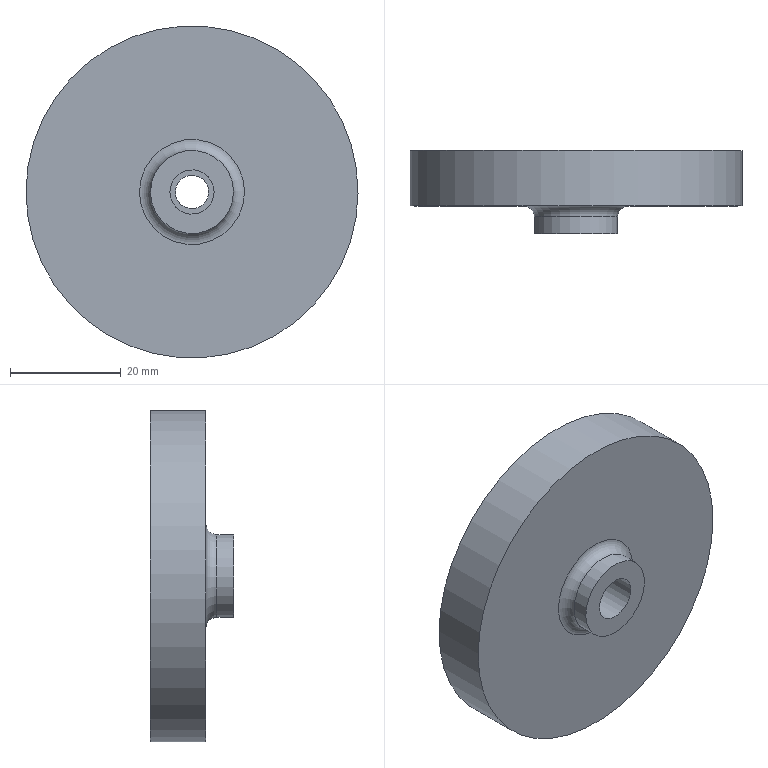Component | NX | PULLEY | 1 solid | 16 faces | box 60 x 15 x 60 mm | volume 22186 mm3 | plane 6 | cylinder 4 | torus 4 | cone 2 | commonest cylinder face diameters 15 x1 60 x1 8 x1 6 x1
STEP:
#1=CARTESIAN_POINT('',(0.,0.,0.));
#2=DIRECTION('',(0.,0.,1.));
#3=DIRECTION('',(1.,0.,0.));
#4=AXIS2_PLACEMENT_3D('',#1,#2,#3);
#5=CARTESIAN_POINT('',(-2.69,59.8,44.627));
#6=VERTEX_POINT('',#5);
#7=CARTESIAN_POINT('',(0.0005589,59.8,43.3));
#8=DIRECTION('',(0.,-1.,0.));
#9=DIRECTION('',(-0.8969,0.,0.4423));
#10=AXIS2_PLACEMENT_3D('',#7,#8,#9);
#11=CIRCLE('',#10,3.);
#12=CARTESIAN_POINT('',(0.0005589,59.8,43.3));
#13=DIRECTION('',(0.,1.,0.));
#14=DIRECTION('',(-0.8969,0.,0.4423));
#15=AXIS2_PLACEMENT_3D('',#12,#13,#14);
#16=PLANE('',#15);
#17=CARTESIAN_POINT('',(3.,-0.));
#18=CARTESIAN_POINT('',(3.,-5.196));
#19=CARTESIAN_POINT('',(-1.5,-2.598));
#20=CARTESIAN_POINT('',(-6.,0.));
#21=CARTESIAN_POINT('',(-1.5,2.598));
#22=CARTESIAN_POINT('',(3.,5.196));
#23=CARTESIAN_POINT('',(3.,-0.));
#24=(BOUNDED_CURVE()B_SPLINE_CURVE(2,(#17,#18,#19,#20,#21,#22,#23),.UNSPECIFIED.,.T.,.F.)B_SPLINE_CURVE_WITH_KNOTS((1,2,2,2,2,1),(-2.094,0.,2.094,4.189,6.283,8.378),.UNSPECIFIED.)CURVE()GEOMETRIC_REPRESENTATION_ITEM()RATIONAL_B_SPLINE_CURVE((1.,0.5,1.,0.5,1.,0.5,1.))REPRESENTATION_ITEM(''));
#25=(GEOMETRIC_REPRESENTATION_CONTEXT(2)PARAMETRIC_REPRESENTATION_CONTEXT()REPRESENTATION_CONTEXT('',''));
#26=DEFINITIONAL_REPRESENTATION('',(#24),#25);
#27=PCURVE('',#16,#26);
#28=CARTESIAN_POINT('',(0.0005589,73.3,43.3));
#29=DIRECTION('',(0.,-1.,0.));
#30=DIRECTION('',(0.8969,0.,-0.4423));
#31=AXIS2_PLACEMENT_3D('',#28,#29,#30);
#32=CYLINDRICAL_SURFACE('',#31,3.);
#33=CARTESIAN_POINT('',(3.142,13.5));
#34=DIRECTION('',(1.,0.));
#35=VECTOR('',#34,1.);
#36=LINE('',#33,#35);
#37=(GEOMETRIC_REPRESENTATION_CONTEXT(2)PARAMETRIC_REPRESENTATION_CONTEXT()REPRESENTATION_CONTEXT('',''));
#38=DEFINITIONAL_REPRESENTATION('',(#36),#37);
#39=PCURVE('',#32,#38);
#40=SURFACE_CURVE('',#11,(#27,#39),.PCURVE_S1.);
#41=EDGE_CURVE('',#6,#6,#40,.T.);
#42=ORIENTED_EDGE('',*,*,#41,.T.);
#43=EDGE_LOOP('',(#42));
#44=FACE_BOUND('',#43,.T.);
#45=CARTESIAN_POINT('',(5.382,59.8,40.646));
#46=VERTEX_POINT('',#45);
#47=CARTESIAN_POINT('',(0.0005589,59.8,43.3));
#48=DIRECTION('',(0.,-1.,0.));
#49=DIRECTION('',(0.8969,0.,-0.4423));
#50=AXIS2_PLACEMENT_3D('',#47,#48,#49);
#51=CIRCLE('',#50,6.);
#52=CARTESIAN_POINT('',(-6.,0.));
#53=CARTESIAN_POINT('',(-6.,10.392));
#54=CARTESIAN_POINT('',(3.,5.196));
#55=CARTESIAN_POINT('',(12.,0.));
#56=CARTESIAN_POINT('',(3.,-5.196));
#57=CARTESIAN_POINT('',(-6.,-10.392));
#58=CARTESIAN_POINT('',(-6.,0.));
#59=(BOUNDED_CURVE()B_SPLINE_CURVE(2,(#52,#53,#54,#55,#56,#57,#58),.UNSPECIFIED.,.T.,.F.)B_SPLINE_CURVE_WITH_KNOTS((1,2,2,2,2,1),(-2.094,0.,2.094,4.189,6.283,8.378),.UNSPECIFIED.)CURVE()GEOMETRIC_REPRESENTATION_ITEM()RATIONAL_B_SPLINE_CURVE((1.,0.5,1.,0.5,1.,0.5,1.))REPRESENTATION_ITEM(''));
#60=(GEOMETRIC_REPRESENTATION_CONTEXT(2)PARAMETRIC_REPRESENTATION_CONTEXT()REPRESENTATION_CONTEXT('',''));
#61=DEFINITIONAL_REPRESENTATION('',(#59),#60);
#62=PCURVE('',#16,#61);
#63=CARTESIAN_POINT('',(0.0005589,53.8,43.3));
#64=DIRECTION('',(0.,-1.,0.));
#65=DIRECTION('',(0.8969,0.,-0.4423));
#66=AXIS2_PLACEMENT_3D('',#63,#64,#65);
#67=CONICAL_SURFACE('',#66,6.843,0.1396);
#68=CARTESIAN_POINT('',(0.,-6.));
#69=DIRECTION('',(1.,-0.));
#70=VECTOR('',#69,1.);
#71=LINE('',#68,#70);
#72=(GEOMETRIC_REPRESENTATION_CONTEXT(2)PARAMETRIC_REPRESENTATION_CONTEXT()REPRESENTATION_CONTEXT('',''));
#73=DEFINITIONAL_REPRESENTATION('',(#71),#72);
#74=PCURVE('',#67,#73);
#75=SURFACE_CURVE('',#51,(#62,#74),.PCURVE_S1.);
#76=EDGE_CURVE('',#46,#46,#75,.T.);
#77=ORIENTED_EDGE('',*,*,#76,.F.);
#78=EDGE_LOOP('',(#77));
#79=FACE_BOUND('',#78,.T.);
#80=ADVANCED_FACE('',(#44,#79),#16,.T.);
#81=CARTESIAN_POINT('',(-3.587,44.8,45.069));
#82=VERTEX_POINT('',#81);
#83=CARTESIAN_POINT('',(0.0005589,44.8,43.3));
#84=DIRECTION('',(0.,1.,0.));
#85=DIRECTION('',(-0.8969,0.,0.4423));
#86=AXIS2_PLACEMENT_3D('',#83,#84,#85);
#87=CIRCLE('',#86,4.);
#88=CARTESIAN_POINT('',(0.0005589,44.8,43.3));
#89=DIRECTION('',(0.,-1.,0.));
#90=DIRECTION('',(0.8969,0.,-0.4423));
#91=AXIS2_PLACEMENT_3D('',#88,#89,#90);
#92=PLANE('',#91);
#93=CARTESIAN_POINT('',(-4.,0.));
#94=CARTESIAN_POINT('',(-4.,6.928));
#95=CARTESIAN_POINT('',(2.,3.464));
#96=CARTESIAN_POINT('',(8.,0.));
#97=CARTESIAN_POINT('',(2.,-3.464));
#98=CARTESIAN_POINT('',(-4.,-6.928));
#99=CARTESIAN_POINT('',(-4.,0.));
#100=(BOUNDED_CURVE()B_SPLINE_CURVE(2,(#93,#94,#95,#96,#97,#98,#99),.UNSPECIFIED.,.T.,.F.)B_SPLINE_CURVE_WITH_KNOTS((1,2,2,2,2,1),(-2.094,0.,2.094,4.189,6.283,8.378),.UNSPECIFIED.)CURVE()GEOMETRIC_REPRESENTATION_ITEM()RATIONAL_B_SPLINE_CURVE((1.,0.5,1.,0.5,1.,0.5,1.))REPRESENTATION_ITEM(''));
#101=(GEOMETRIC_REPRESENTATION_CONTEXT(2)PARAMETRIC_REPRESENTATION_CONTEXT()REPRESENTATION_CONTEXT('',''));
#102=DEFINITIONAL_REPRESENTATION('',(#100),#101);
#103=PCURVE('',#92,#102);
#104=CARTESIAN_POINT('',(0.0005589,52.3,43.3));
#105=DIRECTION('',(0.,-1.,0.));
#106=DIRECTION('',(0.8969,0.,-0.4423));
#107=AXIS2_PLACEMENT_3D('',#104,#105,#106);
#108=CYLINDRICAL_SURFACE('',#107,4.);
#109=CARTESIAN_POINT('',(9.425,7.5));
#110=DIRECTION('',(-1.,0.));
#111=VECTOR('',#110,1.);
#112=LINE('',#109,#111);
#113=(GEOMETRIC_REPRESENTATION_CONTEXT(2)PARAMETRIC_REPRESENTATION_CONTEXT()REPRESENTATION_CONTEXT('',''));
#114=DEFINITIONAL_REPRESENTATION('',(#112),#113);
#115=PCURVE('',#108,#114);
#116=SURFACE_CURVE('',#87,(#103,#115),.PCURVE_S1.);
#117=EDGE_CURVE('',#82,#82,#116,.T.);
#118=ORIENTED_EDGE('',*,*,#117,.T.);
#119=EDGE_LOOP('',(#118));
#120=FACE_BOUND('',#119,.T.);
#121=CARTESIAN_POINT('',(-6.726,44.8,46.617));
#122=VERTEX_POINT('',#121);
#123=CARTESIAN_POINT('',(0.0005589,44.8,43.3));
#124=DIRECTION('',(0.,1.,0.));
#125=DIRECTION('',(-0.8969,0.,0.4423));
#126=AXIS2_PLACEMENT_3D('',#123,#124,#125);
#127=CIRCLE('',#126,7.5);
#128=CARTESIAN_POINT('',(-7.5,0.));
#129=CARTESIAN_POINT('',(-7.5,12.99));
#130=CARTESIAN_POINT('',(3.75,6.495));
#131=CARTESIAN_POINT('',(15.,0.));
#132=CARTESIAN_POINT('',(3.75,-6.495));
#133=CARTESIAN_POINT('',(-7.5,-12.99));
#134=CARTESIAN_POINT('',(-7.5,0.));
#135=(BOUNDED_CURVE()B_SPLINE_CURVE(2,(#128,#129,#130,#131,#132,#133,#134),.UNSPECIFIED.,.T.,.F.)B_SPLINE_CURVE_WITH_KNOTS((1,2,2,2,2,1),(-2.094,0.,2.094,4.189,6.283,8.378),.UNSPECIFIED.)CURVE()GEOMETRIC_REPRESENTATION_ITEM()RATIONAL_B_SPLINE_CURVE((1.,0.5,1.,0.5,1.,0.5,1.))REPRESENTATION_ITEM(''));
#136=(GEOMETRIC_REPRESENTATION_CONTEXT(2)PARAMETRIC_REPRESENTATION_CONTEXT()REPRESENTATION_CONTEXT('',''));
#137=DEFINITIONAL_REPRESENTATION('',(#135),#136);
#138=PCURVE('',#92,#137);
#139=CARTESIAN_POINT('',(0.0005589,44.8,43.3));
#140=DIRECTION('',(0.,1.,0.));
#141=DIRECTION('',(-0.8969,0.,0.4423));
#142=AXIS2_PLACEMENT_3D('',#139,#140,#141);
#143=CYLINDRICAL_SURFACE('',#142,7.5);
#144=CARTESIAN_POINT('',(0.,0.));
#145=DIRECTION('',(1.,0.));
#146=VECTOR('',#145,1.);
#147=LINE('',#144,#146);
#148=(GEOMETRIC_REPRESENTATION_CONTEXT(2)PARAMETRIC_REPRESENTATION_CONTEXT()REPRESENTATION_CONTEXT('',''));
#149=DEFINITIONAL_REPRESENTATION('',(#147),#148);
#150=PCURVE('',#143,#149);
#151=SURFACE_CURVE('',#127,(#138,#150),.PCURVE_S1.);
#152=EDGE_CURVE('',#122,#122,#151,.T.);
#153=ORIENTED_EDGE('',*,*,#152,.F.);
#154=EDGE_LOOP('',(#153));
#155=FACE_BOUND('',#154,.T.);
#156=ADVANCED_FACE('',(#120,#155),#92,.T.);
#157=CARTESIAN_POINT('',(6.727,47.8,39.983));
#158=VERTEX_POINT('',#157);
#159=CARTESIAN_POINT('',(-6.726,47.8,46.617));
#160=VERTEX_POINT('',#159);
#161=CARTESIAN_POINT('',(0.0005589,47.8,43.3));
#162=DIRECTION('',(0.,-1.,0.));
#163=DIRECTION('',(0.8969,0.,-0.4423));
#164=AXIS2_PLACEMENT_3D('',#161,#162,#163);
#165=CIRCLE('',#164,7.5);
#166=CARTESIAN_POINT('',(3.142,3.));
#167=DIRECTION('',(-1.,0.));
#168=VECTOR('',#167,1.);
#169=LINE('',#166,#168);
#170=(GEOMETRIC_REPRESENTATION_CONTEXT(2)PARAMETRIC_REPRESENTATION_CONTEXT()REPRESENTATION_CONTEXT('',''));
#171=DEFINITIONAL_REPRESENTATION('',(#169),#170);
#172=PCURVE('',#143,#171);
#173=CARTESIAN_POINT('',(0.0005589,47.8,43.3));
#174=DIRECTION('',(0.,-1.,0.));
#175=DIRECTION('',(0.8969,0.,-0.4423));
#176=AXIS2_PLACEMENT_3D('',#173,#174,#175);
#177=TOROIDAL_SURFACE('',#176,9.5,2.);
#178=CARTESIAN_POINT('',(0.,3.142));
#179=DIRECTION('',(1.,-0.));
#180=VECTOR('',#179,1.);
#181=LINE('',#178,#180);
#182=(GEOMETRIC_REPRESENTATION_CONTEXT(2)PARAMETRIC_REPRESENTATION_CONTEXT()REPRESENTATION_CONTEXT('',''));
#183=DEFINITIONAL_REPRESENTATION('',(#181),#182);
#184=PCURVE('',#177,#183);
#185=SURFACE_CURVE('',#165,(#172,#184),.PCURVE_S1.);
#186=EDGE_CURVE('',#158,#160,#185,.T.);
#187=ORIENTED_EDGE('',*,*,#186,.T.);
#188=CARTESIAN_POINT('',(-6.726,44.8,46.617));
#189=CARTESIAN_POINT('',(-6.726,47.8,46.617));
#190=B_SPLINE_CURVE_WITH_KNOTS('',1,(#188,#189),.UNSPECIFIED.,.F.,.F.,(2,2),(0.,3.),.PIECEWISE_BEZIER_KNOTS.);
#191=CARTESIAN_POINT('',(0.,0.));
#192=DIRECTION('',(0.,1.));
#193=VECTOR('',#192,1.);
#194=LINE('',#191,#193);
#195=(GEOMETRIC_REPRESENTATION_CONTEXT(2)PARAMETRIC_REPRESENTATION_CONTEXT()REPRESENTATION_CONTEXT('',''));
#196=DEFINITIONAL_REPRESENTATION('',(#194),#195);
#197=PCURVE('',#143,#196);
#198=CARTESIAN_POINT('',(6.283,0.));
#199=DIRECTION('',(0.,1.));
#200=VECTOR('',#199,1.);
#201=LINE('',#198,#200);
#202=(GEOMETRIC_REPRESENTATION_CONTEXT(2)PARAMETRIC_REPRESENTATION_CONTEXT()REPRESENTATION_CONTEXT('',''));
#203=DEFINITIONAL_REPRESENTATION('',(#201),#202);
#204=PCURVE('',#143,#203);
#205=SEAM_CURVE('',#190,(#197,#204),.PCURVE_S1.);
#206=EDGE_CURVE('',#122,#160,#205,.T.);
#207=ORIENTED_EDGE('',*,*,#206,.F.);
#208=ORIENTED_EDGE('',*,*,#152,.T.);
#209=ORIENTED_EDGE('',*,*,#206,.T.);
#210=CARTESIAN_POINT('',(0.0005589,47.8,43.3));
#211=DIRECTION('',(0.,-1.,0.));
#212=DIRECTION('',(0.8969,0.,-0.4423));
#213=AXIS2_PLACEMENT_3D('',#210,#211,#212);
#214=CIRCLE('',#213,7.5);
#215=CARTESIAN_POINT('',(9.425,3.));
#216=DIRECTION('',(-1.,0.));
#217=VECTOR('',#216,1.);
#218=LINE('',#215,#217);
#219=(GEOMETRIC_REPRESENTATION_CONTEXT(2)PARAMETRIC_REPRESENTATION_CONTEXT()REPRESENTATION_CONTEXT('',''));
#220=DEFINITIONAL_REPRESENTATION('',(#218),#219);
#221=PCURVE('',#143,#220);
#222=CARTESIAN_POINT('',(0.,3.142));
#223=DIRECTION('',(1.,0.));
#224=VECTOR('',#223,1.);
#225=LINE('',#222,#224);
#226=(GEOMETRIC_REPRESENTATION_CONTEXT(2)PARAMETRIC_REPRESENTATION_CONTEXT()REPRESENTATION_CONTEXT('',''));
#227=DEFINITIONAL_REPRESENTATION('',(#225),#226);
#228=PCURVE('',#177,#227);
#229=SURFACE_CURVE('',#214,(#221,#228),.PCURVE_S1.);
#230=EDGE_CURVE('',#160,#158,#229,.T.);
#231=ORIENTED_EDGE('',*,*,#230,.T.);
#232=EDGE_LOOP('',(#187,#207,#208,#209,#231));
#233=FACE_BOUND('',#232,.T.);
#234=ADVANCED_FACE('',(#233),#143,.T.);
#235=CARTESIAN_POINT('',(-18.907,59.8,52.624));
#236=VERTEX_POINT('',#235);
#237=CARTESIAN_POINT('',(0.0005589,59.8,43.3));
#238=DIRECTION('',(0.,-1.,0.));
#239=DIRECTION('',(-0.8969,0.,0.4423));
#240=AXIS2_PLACEMENT_3D('',#237,#238,#239);
#241=CIRCLE('',#240,21.081);
#242=CARTESIAN_POINT('',(0.0005589,59.8,43.3));
#243=DIRECTION('',(0.,1.,0.));
#244=DIRECTION('',(-0.8969,0.,0.4423));
#245=AXIS2_PLACEMENT_3D('',#242,#243,#244);
#246=PLANE('',#245);
#247=CARTESIAN_POINT('',(21.081,0.));
#248=CARTESIAN_POINT('',(21.081,-36.514));
#249=CARTESIAN_POINT('',(-10.541,-18.257));
#250=CARTESIAN_POINT('',(-42.163,-0.));
#251=CARTESIAN_POINT('',(-10.541,18.257));
#252=CARTESIAN_POINT('',(21.081,36.514));
#253=CARTESIAN_POINT('',(21.081,0.));
#254=(BOUNDED_CURVE()B_SPLINE_CURVE(2,(#247,#248,#249,#250,#251,#252,#253),.UNSPECIFIED.,.T.,.F.)B_SPLINE_CURVE_WITH_KNOTS((1,2,2,2,2,1),(-2.094,0.,2.094,4.189,6.283,8.378),.UNSPECIFIED.)CURVE()GEOMETRIC_REPRESENTATION_ITEM()RATIONAL_B_SPLINE_CURVE((1.,0.5,1.,0.5,1.,0.5,1.))REPRESENTATION_ITEM(''));
#255=(GEOMETRIC_REPRESENTATION_CONTEXT(2)PARAMETRIC_REPRESENTATION_CONTEXT()REPRESENTATION_CONTEXT('',''));
#256=DEFINITIONAL_REPRESENTATION('',(#254),#255);
#257=PCURVE('',#246,#256);
#258=CARTESIAN_POINT('',(0.0005589,58.8,43.3));
#259=DIRECTION('',(0.,1.,0.));
#260=DIRECTION('',(-0.8969,0.,0.4423));
#261=AXIS2_PLACEMENT_3D('',#258,#259,#260);
#262=TOROIDAL_SURFACE('',#261,21.081,1.);
#263=CARTESIAN_POINT('',(6.283,7.854));
#264=DIRECTION('',(-1.,0.));
#265=VECTOR('',#264,1.);
#266=LINE('',#263,#265);
#267=(GEOMETRIC_REPRESENTATION_CONTEXT(2)PARAMETRIC_REPRESENTATION_CONTEXT()REPRESENTATION_CONTEXT('',''));
#268=DEFINITIONAL_REPRESENTATION('',(#266),#267);
#269=PCURVE('',#262,#268);
#270=SURFACE_CURVE('',#241,(#257,#269),.PCURVE_S1.);
#271=EDGE_CURVE('',#236,#236,#270,.T.);
#272=ORIENTED_EDGE('',*,*,#271,.T.);
#273=EDGE_LOOP('',(#272));
#274=FACE_BOUND('',#273,.T.);
#275=CARTESIAN_POINT('',(-26.906,59.8,56.569));
#276=VERTEX_POINT('',#275);
#277=CARTESIAN_POINT('',(0.0005589,59.8,43.3));
#278=DIRECTION('',(0.,1.,0.));
#279=DIRECTION('',(-0.8969,0.,0.4423));
#280=AXIS2_PLACEMENT_3D('',#277,#278,#279);
#281=CIRCLE('',#280,30.);
#282=CARTESIAN_POINT('',(0.,0.));
#283=DIRECTION('',(1.,0.));
#284=AXIS2_PLACEMENT_2D('',#282,#283);
#285=CIRCLE('',#284,30.);
#286=(GEOMETRIC_REPRESENTATION_CONTEXT(2)PARAMETRIC_REPRESENTATION_CONTEXT()REPRESENTATION_CONTEXT('',''));
#287=DEFINITIONAL_REPRESENTATION('',(#285),#286);
#288=PCURVE('',#246,#287);
#289=CARTESIAN_POINT('',(0.0005589,49.8,43.3));
#290=DIRECTION('',(0.,1.,0.));
#291=DIRECTION('',(-0.8969,0.,0.4423));
#292=AXIS2_PLACEMENT_3D('',#289,#290,#291);
#293=CYLINDRICAL_SURFACE('',#292,30.);
#294=CARTESIAN_POINT('',(0.,10.));
#295=DIRECTION('',(1.,0.));
#296=VECTOR('',#295,1.);
#297=LINE('',#294,#296);
#298=(GEOMETRIC_REPRESENTATION_CONTEXT(2)PARAMETRIC_REPRESENTATION_CONTEXT()REPRESENTATION_CONTEXT('',''));
#299=DEFINITIONAL_REPRESENTATION('',(#297),#298);
#300=PCURVE('',#293,#299);
#301=SURFACE_CURVE('',#281,(#288,#300),.PCURVE_S1.);
#302=EDGE_CURVE('',#276,#276,#301,.T.);
#303=ORIENTED_EDGE('',*,*,#302,.T.);
#304=EDGE_LOOP('',(#303));
#305=FACE_BOUND('',#304,.T.);
#306=ADVANCED_FACE('',(#274,#305),#246,.T.);
#307=CARTESIAN_POINT('',(8.521,49.8,39.098));
#308=VERTEX_POINT('',#307);
#309=CARTESIAN_POINT('',(0.0005589,49.8,43.3));
#310=DIRECTION('',(0.,1.,0.));
#311=DIRECTION('',(0.8969,0.,-0.4423));
#312=AXIS2_PLACEMENT_3D('',#309,#310,#311);
#313=CIRCLE('',#312,9.5);
#314=CARTESIAN_POINT('',(0.0005589,49.8,43.3));
#315=DIRECTION('',(0.,-1.,0.));
#316=DIRECTION('',(0.8969,0.,-0.4423));
#317=AXIS2_PLACEMENT_3D('',#314,#315,#316);
#318=PLANE('',#317);
#319=CARTESIAN_POINT('',(9.5,-0.));
#320=CARTESIAN_POINT('',(9.5,-16.454));
#321=CARTESIAN_POINT('',(-4.75,-8.227));
#322=CARTESIAN_POINT('',(-19.,0.));
#323=CARTESIAN_POINT('',(-4.75,8.227));
#324=CARTESIAN_POINT('',(9.5,16.454));
#325=CARTESIAN_POINT('',(9.5,-0.));
#326=(BOUNDED_CURVE()B_SPLINE_CURVE(2,(#319,#320,#321,#322,#323,#324,#325),.UNSPECIFIED.,.T.,.F.)B_SPLINE_CURVE_WITH_KNOTS((1,2,2,2,2,1),(-2.094,0.,2.094,4.189,6.283,8.378),.UNSPECIFIED.)CURVE()GEOMETRIC_REPRESENTATION_ITEM()RATIONAL_B_SPLINE_CURVE((1.,0.5,1.,0.5,1.,0.5,1.))REPRESENTATION_ITEM(''));
#327=(GEOMETRIC_REPRESENTATION_CONTEXT(2)PARAMETRIC_REPRESENTATION_CONTEXT()REPRESENTATION_CONTEXT('',''));
#328=DEFINITIONAL_REPRESENTATION('',(#326),#327);
#329=PCURVE('',#318,#328);
#330=CARTESIAN_POINT('',(6.283,4.712));
#331=DIRECTION('',(-1.,0.));
#332=VECTOR('',#331,1.);
#333=LINE('',#330,#332);
#334=(GEOMETRIC_REPRESENTATION_CONTEXT(2)PARAMETRIC_REPRESENTATION_CONTEXT()REPRESENTATION_CONTEXT('',''));
#335=DEFINITIONAL_REPRESENTATION('',(#333),#334);
#336=PCURVE('',#177,#335);
#337=SURFACE_CURVE('',#313,(#329,#336),.PCURVE_S1.);
#338=EDGE_CURVE('',#308,#308,#337,.T.);
#339=ORIENTED_EDGE('',*,*,#338,.T.);
#340=EDGE_LOOP('',(#339));
#341=FACE_BOUND('',#340,.T.);
#342=CARTESIAN_POINT('',(-26.906,49.8,56.569));
#343=VERTEX_POINT('',#342);
#344=CARTESIAN_POINT('',(0.0005589,49.8,43.3));
#345=DIRECTION('',(0.,1.,0.));
#346=DIRECTION('',(-0.8969,0.,0.4423));
#347=AXIS2_PLACEMENT_3D('',#344,#345,#346);
#348=CIRCLE('',#347,30.);
#349=CARTESIAN_POINT('',(-30.,0.));
#350=CARTESIAN_POINT('',(-30.,51.962));
#351=CARTESIAN_POINT('',(15.,25.981));
#352=CARTESIAN_POINT('',(60.,0.));
#353=CARTESIAN_POINT('',(15.,-25.981));
#354=CARTESIAN_POINT('',(-30.,-51.962));
#355=CARTESIAN_POINT('',(-30.,0.));
#356=(BOUNDED_CURVE()B_SPLINE_CURVE(2,(#349,#350,#351,#352,#353,#354,#355),.UNSPECIFIED.,.T.,.F.)B_SPLINE_CURVE_WITH_KNOTS((1,2,2,2,2,1),(-2.094,0.,2.094,4.189,6.283,8.378),.UNSPECIFIED.)CURVE()GEOMETRIC_REPRESENTATION_ITEM()RATIONAL_B_SPLINE_CURVE((1.,0.5,1.,0.5,1.,0.5,1.))REPRESENTATION_ITEM(''));
#357=(GEOMETRIC_REPRESENTATION_CONTEXT(2)PARAMETRIC_REPRESENTATION_CONTEXT()REPRESENTATION_CONTEXT('',''));
#358=DEFINITIONAL_REPRESENTATION('',(#356),#357);
#359=PCURVE('',#318,#358);
#360=CARTESIAN_POINT('',(0.,0.));
#361=DIRECTION('',(1.,0.));
#362=VECTOR('',#361,1.);
#363=LINE('',#360,#362);
#364=(GEOMETRIC_REPRESENTATION_CONTEXT(2)PARAMETRIC_REPRESENTATION_CONTEXT()REPRESENTATION_CONTEXT('',''));
#365=DEFINITIONAL_REPRESENTATION('',(#363),#364);
#366=PCURVE('',#293,#365);
#367=SURFACE_CURVE('',#348,(#359,#366),.PCURVE_S1.);
#368=EDGE_CURVE('',#343,#343,#367,.T.);
#369=ORIENTED_EDGE('',*,*,#368,.F.);
#370=EDGE_LOOP('',(#369));
#371=FACE_BOUND('',#370,.T.);
#372=ADVANCED_FACE('',(#341,#371),#318,.T.);
#373=ORIENTED_EDGE('',*,*,#302,.F.);
#374=CARTESIAN_POINT('',(-26.906,49.8,56.569));
#375=CARTESIAN_POINT('',(-26.906,59.8,56.569));
#376=B_SPLINE_CURVE_WITH_KNOTS('',1,(#374,#375),.UNSPECIFIED.,.F.,.F.,(2,2),(0.,10.),.PIECEWISE_BEZIER_KNOTS.);
#377=CARTESIAN_POINT('',(0.,0.));
#378=DIRECTION('',(0.,1.));
#379=VECTOR('',#378,1.);
#380=LINE('',#377,#379);
#381=(GEOMETRIC_REPRESENTATION_CONTEXT(2)PARAMETRIC_REPRESENTATION_CONTEXT()REPRESENTATION_CONTEXT('',''));
#382=DEFINITIONAL_REPRESENTATION('',(#380),#381);
#383=PCURVE('',#293,#382);
#384=CARTESIAN_POINT('',(6.283,0.));
#385=DIRECTION('',(0.,1.));
#386=VECTOR('',#385,1.);
#387=LINE('',#384,#386);
#388=(GEOMETRIC_REPRESENTATION_CONTEXT(2)PARAMETRIC_REPRESENTATION_CONTEXT()REPRESENTATION_CONTEXT('',''));
#389=DEFINITIONAL_REPRESENTATION('',(#387),#388);
#390=PCURVE('',#293,#389);
#391=SEAM_CURVE('',#376,(#383,#390),.PCURVE_S1.);
#392=EDGE_CURVE('',#343,#276,#391,.T.);
#393=ORIENTED_EDGE('',*,*,#392,.F.);
#394=ORIENTED_EDGE('',*,*,#368,.T.);
#395=ORIENTED_EDGE('',*,*,#392,.T.);
#396=EDGE_LOOP('',(#373,#393,#394,#395));
#397=FACE_BOUND('',#396,.T.);
#398=ADVANCED_FACE('',(#397),#293,.T.);
#399=CARTESIAN_POINT('',(-3.587,52.3,45.069));
#400=VERTEX_POINT('',#399);
#401=CARTESIAN_POINT('',(0.0005589,52.3,43.3));
#402=DIRECTION('',(0.,-1.,0.));
#403=DIRECTION('',(-0.8969,0.,0.4423));
#404=AXIS2_PLACEMENT_3D('',#401,#402,#403);
#405=CIRCLE('',#404,4.);
#406=CARTESIAN_POINT('',(3.142,0.));
#407=DIRECTION('',(1.,0.));
#408=VECTOR('',#407,1.);
#409=LINE('',#406,#408);
#410=(GEOMETRIC_REPRESENTATION_CONTEXT(2)PARAMETRIC_REPRESENTATION_CONTEXT()REPRESENTATION_CONTEXT('',''));
#411=DEFINITIONAL_REPRESENTATION('',(#409),#410);
#412=PCURVE('',#108,#411);
#413=CARTESIAN_POINT('',(0.0005589,52.3,43.3));
#414=DIRECTION('',(0.,1.,0.));
#415=DIRECTION('',(-0.8969,0.,0.4423));
#416=AXIS2_PLACEMENT_3D('',#413,#414,#415);
#417=PLANE('',#416);
#418=CARTESIAN_POINT('',(4.,0.));
#419=CARTESIAN_POINT('',(4.,-6.928));
#420=CARTESIAN_POINT('',(-2.,-3.464));
#421=CARTESIAN_POINT('',(-8.,-0.));
#422=CARTESIAN_POINT('',(-2.,3.464));
#423=CARTESIAN_POINT('',(4.,6.928));
#424=CARTESIAN_POINT('',(4.,0.));
#425=(BOUNDED_CURVE()B_SPLINE_CURVE(2,(#418,#419,#420,#421,#422,#423,#424),.UNSPECIFIED.,.T.,.F.)B_SPLINE_CURVE_WITH_KNOTS((1,2,2,2,2,1),(-2.094,0.,2.094,4.189,6.283,8.378),.UNSPECIFIED.)CURVE()GEOMETRIC_REPRESENTATION_ITEM()RATIONAL_B_SPLINE_CURVE((1.,0.5,1.,0.5,1.,0.5,1.))REPRESENTATION_ITEM(''));
#426=(GEOMETRIC_REPRESENTATION_CONTEXT(2)PARAMETRIC_REPRESENTATION_CONTEXT()REPRESENTATION_CONTEXT('',''));
#427=DEFINITIONAL_REPRESENTATION('',(#425),#426);
#428=PCURVE('',#417,#427);
#429=SURFACE_CURVE('',#405,(#412,#428),.PCURVE_S1.);
#430=EDGE_CURVE('',#400,#400,#429,.T.);
#431=ORIENTED_EDGE('',*,*,#430,.T.);
#432=CARTESIAN_POINT('',(-3.587,52.3,45.069));
#433=CARTESIAN_POINT('',(-3.587,44.8,45.069));
#434=B_SPLINE_CURVE_WITH_KNOTS('',1,(#432,#433),.UNSPECIFIED.,.F.,.F.,(2,2),(0.,7.5),.PIECEWISE_BEZIER_KNOTS.);
#435=CARTESIAN_POINT('',(9.425,0.));
#436=DIRECTION('',(0.,1.));
#437=VECTOR('',#436,1.);
#438=LINE('',#435,#437);
#439=(GEOMETRIC_REPRESENTATION_CONTEXT(2)PARAMETRIC_REPRESENTATION_CONTEXT()REPRESENTATION_CONTEXT('',''));
#440=DEFINITIONAL_REPRESENTATION('',(#438),#439);
#441=PCURVE('',#108,#440);
#442=CARTESIAN_POINT('',(3.142,0.));
#443=DIRECTION('',(0.,1.));
#444=VECTOR('',#443,1.);
#445=LINE('',#442,#444);
#446=(GEOMETRIC_REPRESENTATION_CONTEXT(2)PARAMETRIC_REPRESENTATION_CONTEXT()REPRESENTATION_CONTEXT('',''));
#447=DEFINITIONAL_REPRESENTATION('',(#445),#446);
#448=PCURVE('',#108,#447);
#449=SEAM_CURVE('',#434,(#441,#448),.PCURVE_S1.);
#450=EDGE_CURVE('',#400,#82,#449,.T.);
#451=ORIENTED_EDGE('',*,*,#450,.T.);
#452=ORIENTED_EDGE('',*,*,#117,.T.);
#453=ORIENTED_EDGE('',*,*,#450,.F.);
#454=EDGE_LOOP('',(#431,#451,#452,#453));
#455=FACE_BOUND('',#454,.F.);
#456=ADVANCED_FACE('',(#455),#108,.F.);
#457=CARTESIAN_POINT('',(-2.69,52.3,44.627));
#458=VERTEX_POINT('',#457);
#459=CARTESIAN_POINT('',(0.0005589,52.3,43.3));
#460=DIRECTION('',(0.,1.,0.));
#461=DIRECTION('',(-0.8969,0.,0.4423));
#462=AXIS2_PLACEMENT_3D('',#459,#460,#461);
#463=CIRCLE('',#462,3.);
#464=CARTESIAN_POINT('',(0.,0.));
#465=DIRECTION('',(1.,-0.));
#466=AXIS2_PLACEMENT_2D('',#464,#465);
#467=CIRCLE('',#466,3.);
#468=(GEOMETRIC_REPRESENTATION_CONTEXT(2)PARAMETRIC_REPRESENTATION_CONTEXT()REPRESENTATION_CONTEXT('',''));
#469=DEFINITIONAL_REPRESENTATION('',(#467),#468);
#470=PCURVE('',#417,#469);
#471=CARTESIAN_POINT('',(9.425,21.));
#472=DIRECTION('',(-1.,0.));
#473=VECTOR('',#472,1.);
#474=LINE('',#471,#473);
#475=(GEOMETRIC_REPRESENTATION_CONTEXT(2)PARAMETRIC_REPRESENTATION_CONTEXT()REPRESENTATION_CONTEXT('',''));
#476=DEFINITIONAL_REPRESENTATION('',(#474),#475);
#477=PCURVE('',#32,#476);
#478=SURFACE_CURVE('',#463,(#470,#477),.PCURVE_S1.);
#479=EDGE_CURVE('',#458,#458,#478,.T.);
#480=ORIENTED_EDGE('',*,*,#479,.T.);
#481=EDGE_LOOP('',(#480));
#482=FACE_BOUND('',#481,.T.);
#483=ORIENTED_EDGE('',*,*,#430,.T.);
#484=EDGE_LOOP('',(#483));
#485=FACE_BOUND('',#484,.T.);
#486=ADVANCED_FACE('',(#482,#485),#417,.F.);
#487=ORIENTED_EDGE('',*,*,#41,.T.);
#488=CARTESIAN_POINT('',(-2.69,59.8,44.627));
#489=CARTESIAN_POINT('',(-2.69,52.3,44.627));
#490=B_SPLINE_CURVE_WITH_KNOTS('',1,(#488,#489),.UNSPECIFIED.,.F.,.F.,(2,2),(13.5,21.),.PIECEWISE_BEZIER_KNOTS.);
#491=CARTESIAN_POINT('',(9.425,0.));
#492=DIRECTION('',(0.,1.));
#493=VECTOR('',#492,1.);
#494=LINE('',#491,#493);
#495=(GEOMETRIC_REPRESENTATION_CONTEXT(2)PARAMETRIC_REPRESENTATION_CONTEXT()REPRESENTATION_CONTEXT('',''));
#496=DEFINITIONAL_REPRESENTATION('',(#494),#495);
#497=PCURVE('',#32,#496);
#498=CARTESIAN_POINT('',(3.142,0.));
#499=DIRECTION('',(0.,1.));
#500=VECTOR('',#499,1.);
#501=LINE('',#498,#500);
#502=(GEOMETRIC_REPRESENTATION_CONTEXT(2)PARAMETRIC_REPRESENTATION_CONTEXT()REPRESENTATION_CONTEXT('',''));
#503=DEFINITIONAL_REPRESENTATION('',(#501),#502);
#504=PCURVE('',#32,#503);
#505=SEAM_CURVE('',#490,(#497,#504),.PCURVE_S1.);
#506=EDGE_CURVE('',#6,#458,#505,.T.);
#507=ORIENTED_EDGE('',*,*,#506,.T.);
#508=ORIENTED_EDGE('',*,*,#479,.T.);
#509=ORIENTED_EDGE('',*,*,#506,.F.);
#510=EDGE_LOOP('',(#487,#507,#508,#509));
#511=FACE_BOUND('',#510,.F.);
#512=ADVANCED_FACE('',(#511),#32,.F.);
#513=CARTESIAN_POINT('',(-18.036,59.042,52.195));
#514=VERTEX_POINT('',#513);
#515=CARTESIAN_POINT('',(18.037,59.042,34.405));
#516=VERTEX_POINT('',#515);
#517=CARTESIAN_POINT('',(0.0005589,59.042,43.3));
#518=DIRECTION('',(0.,1.,0.));
#519=DIRECTION('',(0.8969,0.,-0.4423));
#520=AXIS2_PLACEMENT_3D('',#517,#518,#519);
#521=CIRCLE('',#520,20.111);
#522=CARTESIAN_POINT('',(0.0005589,59.8,43.3));
#523=DIRECTION('',(0.,1.,0.));
#524=DIRECTION('',(-0.8969,0.,0.4423));
#525=AXIS2_PLACEMENT_3D('',#522,#523,#524);
#526=CONICAL_SURFACE('',#525,20.3,0.2443);
#527=CARTESIAN_POINT('',(-3.142,-0.7581));
#528=DIRECTION('',(1.,0.));
#529=VECTOR('',#528,1.);
#530=LINE('',#527,#529);
#531=(GEOMETRIC_REPRESENTATION_CONTEXT(2)PARAMETRIC_REPRESENTATION_CONTEXT()REPRESENTATION_CONTEXT('',''));
#532=DEFINITIONAL_REPRESENTATION('',(#530),#531);
#533=PCURVE('',#526,#532);
#534=CARTESIAN_POINT('',(-3.142,9.18));
#535=DIRECTION('',(1.,-0.));
#536=VECTOR('',#535,1.);
#537=LINE('',#534,#536);
#538=(GEOMETRIC_REPRESENTATION_CONTEXT(2)PARAMETRIC_REPRESENTATION_CONTEXT()REPRESENTATION_CONTEXT('',''));
#539=DEFINITIONAL_REPRESENTATION('',(#537),#538);
#540=PCURVE('',#262,#539);
#541=SURFACE_CURVE('',#521,(#533,#540),.PCURVE_S1.);
#542=EDGE_CURVE('',#514,#516,#541,.T.);
#543=ORIENTED_EDGE('',*,*,#542,.F.);
#544=CARTESIAN_POINT('',(-17.034,54.558,51.701));
#545=VERTEX_POINT('',#544);
#546=CARTESIAN_POINT('',(-17.034,54.558,51.701));
#547=CARTESIAN_POINT('',(-18.036,59.042,52.195));
#548=B_SPLINE_CURVE_WITH_KNOTS('',1,(#546,#547),.UNSPECIFIED.,.F.,.F.,(2,2),(-5.402,-0.7813),.PIECEWISE_BEZIER_KNOTS.);
#549=CARTESIAN_POINT('',(0.,0.));
#550=DIRECTION('',(0.,1.));
#551=VECTOR('',#550,1.);
#552=LINE('',#549,#551);
#553=(GEOMETRIC_REPRESENTATION_CONTEXT(2)PARAMETRIC_REPRESENTATION_CONTEXT()REPRESENTATION_CONTEXT('',''));
#554=DEFINITIONAL_REPRESENTATION('',(#552),#553);
#555=PCURVE('',#526,#554);
#556=CARTESIAN_POINT('',(6.283,0.));
#557=DIRECTION('',(0.,1.));
#558=VECTOR('',#557,1.);
#559=LINE('',#556,#558);
#560=(GEOMETRIC_REPRESENTATION_CONTEXT(2)PARAMETRIC_REPRESENTATION_CONTEXT()REPRESENTATION_CONTEXT('',''));
#561=DEFINITIONAL_REPRESENTATION('',(#559),#560);
#562=PCURVE('',#526,#561);
#563=SEAM_CURVE('',#548,(#555,#562),.PCURVE_S1.);
#564=EDGE_CURVE('',#545,#514,#563,.T.);
#565=ORIENTED_EDGE('',*,*,#564,.F.);
#566=CARTESIAN_POINT('',(0.0005589,54.558,43.3));
#567=DIRECTION('',(0.,-1.,0.));
#568=DIRECTION('',(-0.8969,0.,0.4423));
#569=AXIS2_PLACEMENT_3D('',#566,#567,#568);
#570=CIRCLE('',#569,18.993);
#571=CARTESIAN_POINT('',(6.283,-5.242));
#572=DIRECTION('',(-1.,-0.));
#573=VECTOR('',#572,1.);
#574=LINE('',#571,#573);
#575=(GEOMETRIC_REPRESENTATION_CONTEXT(2)PARAMETRIC_REPRESENTATION_CONTEXT()REPRESENTATION_CONTEXT('',''));
#576=DEFINITIONAL_REPRESENTATION('',(#574),#575);
#577=PCURVE('',#526,#576);
#578=CARTESIAN_POINT('',(0.0005589,54.8,43.3));
#579=DIRECTION('',(0.,1.,0.));
#580=DIRECTION('',(-0.8969,0.,0.4423));
#581=AXIS2_PLACEMENT_3D('',#578,#579,#580);
#582=TOROIDAL_SURFACE('',#581,18.023,1.);
#583=CARTESIAN_POINT('',(6.283,6.039));
#584=DIRECTION('',(-1.,-0.));
#585=VECTOR('',#584,1.);
#586=LINE('',#583,#585);
#587=(GEOMETRIC_REPRESENTATION_CONTEXT(2)PARAMETRIC_REPRESENTATION_CONTEXT()REPRESENTATION_CONTEXT('',''));
#588=DEFINITIONAL_REPRESENTATION('',(#586),#587);
#589=PCURVE('',#582,#588);
#590=SURFACE_CURVE('',#570,(#577,#589),.PCURVE_S1.);
#591=EDGE_CURVE('',#545,#545,#590,.T.);
#592=ORIENTED_EDGE('',*,*,#591,.F.);
#593=ORIENTED_EDGE('',*,*,#564,.T.);
#594=CARTESIAN_POINT('',(0.0005589,59.042,43.3));
#595=DIRECTION('',(0.,1.,0.));
#596=DIRECTION('',(0.8969,0.,-0.4423));
#597=AXIS2_PLACEMENT_3D('',#594,#595,#596);
#598=CIRCLE('',#597,20.111);
#599=CARTESIAN_POINT('',(3.142,-0.7581));
#600=DIRECTION('',(1.,0.));
#601=VECTOR('',#600,1.);
#602=LINE('',#599,#601);
#603=(GEOMETRIC_REPRESENTATION_CONTEXT(2)PARAMETRIC_REPRESENTATION_CONTEXT()REPRESENTATION_CONTEXT('',''));
#604=DEFINITIONAL_REPRESENTATION('',(#602),#603);
#605=PCURVE('',#526,#604);
#606=CARTESIAN_POINT('',(3.142,9.18));
#607=DIRECTION('',(1.,0.));
#608=VECTOR('',#607,1.);
#609=LINE('',#606,#608);
#610=(GEOMETRIC_REPRESENTATION_CONTEXT(2)PARAMETRIC_REPRESENTATION_CONTEXT()REPRESENTATION_CONTEXT('',''));
#611=DEFINITIONAL_REPRESENTATION('',(#609),#610);
#612=PCURVE('',#262,#611);
#613=SURFACE_CURVE('',#598,(#605,#612),.PCURVE_S1.);
#614=EDGE_CURVE('',#516,#514,#613,.T.);
#615=ORIENTED_EDGE('',*,*,#614,.F.);
#616=EDGE_LOOP('',(#543,#565,#592,#593,#615));
#617=FACE_BOUND('',#616,.F.);
#618=ADVANCED_FACE('',(#617),#526,.F.);
#619=CARTESIAN_POINT('',(-6.917,53.8,46.711));
#620=VERTEX_POINT('',#619);
#621=CARTESIAN_POINT('',(0.0005589,53.8,43.3));
#622=DIRECTION('',(0.,-1.,0.));
#623=DIRECTION('',(-0.8969,0.,0.4423));
#624=AXIS2_PLACEMENT_3D('',#621,#622,#623);
#625=CIRCLE('',#624,7.713);
#626=CARTESIAN_POINT('',(16.865,53.8,34.983));
#627=DIRECTION('',(0.,1.,0.));
#628=DIRECTION('',(-0.8969,0.,0.4423));
#629=AXIS2_PLACEMENT_3D('',#626,#627,#628);
#630=PLANE('',#629);
#631=CARTESIAN_POINT('',(26.517,0.));
#632=CARTESIAN_POINT('',(26.517,-13.358));
#633=CARTESIAN_POINT('',(14.948,-6.679));
#634=CARTESIAN_POINT('',(3.379,0.));
#635=CARTESIAN_POINT('',(14.948,6.679));
#636=CARTESIAN_POINT('',(26.517,13.358));
#637=CARTESIAN_POINT('',(26.517,0.));
#638=(BOUNDED_CURVE()B_SPLINE_CURVE(2,(#631,#632,#633,#634,#635,#636,#637),.UNSPECIFIED.,.T.,.F.)B_SPLINE_CURVE_WITH_KNOTS((1,2,2,2,2,1),(-2.094,0.,2.094,4.189,6.283,8.378),.UNSPECIFIED.)CURVE()GEOMETRIC_REPRESENTATION_ITEM()RATIONAL_B_SPLINE_CURVE((1.,0.5,1.,0.5,1.,0.5,1.))REPRESENTATION_ITEM(''));
#639=(GEOMETRIC_REPRESENTATION_CONTEXT(2)PARAMETRIC_REPRESENTATION_CONTEXT()REPRESENTATION_CONTEXT('',''));
#640=DEFINITIONAL_REPRESENTATION('',(#638),#639);
#641=PCURVE('',#630,#640);
#642=CARTESIAN_POINT('',(0.0005589,54.8,43.3));
#643=DIRECTION('',(0.,1.,0.));
#644=DIRECTION('',(-0.8969,0.,0.4423));
#645=AXIS2_PLACEMENT_3D('',#642,#643,#644);
#646=TOROIDAL_SURFACE('',#645,7.713,1.);
#647=CARTESIAN_POINT('',(6.283,4.712));
#648=DIRECTION('',(-1.,0.));
#649=VECTOR('',#648,1.);
#650=LINE('',#647,#649);
#651=(GEOMETRIC_REPRESENTATION_CONTEXT(2)PARAMETRIC_REPRESENTATION_CONTEXT()REPRESENTATION_CONTEXT('',''));
#652=DEFINITIONAL_REPRESENTATION('',(#650),#651);
#653=PCURVE('',#646,#652);
#654=SURFACE_CURVE('',#625,(#641,#653),.PCURVE_S1.);
#655=EDGE_CURVE('',#620,#620,#654,.T.);
#656=ORIENTED_EDGE('',*,*,#655,.T.);
#657=EDGE_LOOP('',(#656));
#658=FACE_BOUND('',#657,.T.);
#659=CARTESIAN_POINT('',(-16.163,53.8,51.271));
#660=VERTEX_POINT('',#659);
#661=CARTESIAN_POINT('',(0.0005589,53.8,43.3));
#662=DIRECTION('',(0.,1.,0.));
#663=DIRECTION('',(-0.8969,0.,0.4423));
#664=AXIS2_PLACEMENT_3D('',#661,#662,#663);
#665=CIRCLE('',#664,18.023);
#666=CARTESIAN_POINT('',(18.804,0.));
#667=DIRECTION('',(1.,0.));
#668=AXIS2_PLACEMENT_2D('',#666,#667);
#669=CIRCLE('',#668,18.023);
#670=(GEOMETRIC_REPRESENTATION_CONTEXT(2)PARAMETRIC_REPRESENTATION_CONTEXT()REPRESENTATION_CONTEXT('',''));
#671=DEFINITIONAL_REPRESENTATION('',(#669),#670);
#672=PCURVE('',#630,#671);
#673=CARTESIAN_POINT('',(0.,4.712));
#674=DIRECTION('',(1.,0.));
#675=VECTOR('',#674,1.);
#676=LINE('',#673,#675);
#677=(GEOMETRIC_REPRESENTATION_CONTEXT(2)PARAMETRIC_REPRESENTATION_CONTEXT()REPRESENTATION_CONTEXT('',''));
#678=DEFINITIONAL_REPRESENTATION('',(#676),#677);
#679=PCURVE('',#582,#678);
#680=SURFACE_CURVE('',#665,(#672,#679),.PCURVE_S1.);
#681=EDGE_CURVE('',#660,#660,#680,.T.);
#682=ORIENTED_EDGE('',*,*,#681,.T.);
#683=EDGE_LOOP('',(#682));
#684=FACE_BOUND('',#683,.T.);
#685=ADVANCED_FACE('',(#658,#684),#630,.T.);
#686=CARTESIAN_POINT('',(6.03,54.661,40.327));
#687=VERTEX_POINT('',#686);
#688=CARTESIAN_POINT('',(-6.028,54.661,46.273));
#689=VERTEX_POINT('',#688);
#690=CARTESIAN_POINT('',(0.0005589,54.661,43.3));
#691=DIRECTION('',(0.,1.,0.));
#692=DIRECTION('',(0.8969,0.,-0.4423));
#693=AXIS2_PLACEMENT_3D('',#690,#691,#692);
#694=CIRCLE('',#693,6.722);
#695=CARTESIAN_POINT('',(6.283,-0.8608));
#696=DIRECTION('',(-1.,0.));
#697=VECTOR('',#696,1.);
#698=LINE('',#695,#697);
#699=(GEOMETRIC_REPRESENTATION_CONTEXT(2)PARAMETRIC_REPRESENTATION_CONTEXT()REPRESENTATION_CONTEXT('',''));
#700=DEFINITIONAL_REPRESENTATION('',(#698),#699);
#701=PCURVE('',#67,#700);
#702=CARTESIAN_POINT('',(3.142,3.281));
#703=DIRECTION('',(1.,0.));
#704=VECTOR('',#703,1.);
#705=LINE('',#702,#704);
#706=(GEOMETRIC_REPRESENTATION_CONTEXT(2)PARAMETRIC_REPRESENTATION_CONTEXT()REPRESENTATION_CONTEXT('',''));
#707=DEFINITIONAL_REPRESENTATION('',(#705),#706);
#708=PCURVE('',#646,#707);
#709=SURFACE_CURVE('',#694,(#701,#708),.PCURVE_S1.);
#710=EDGE_CURVE('',#687,#689,#709,.T.);
#711=ORIENTED_EDGE('',*,*,#710,.T.);
#712=CARTESIAN_POINT('',(0.0005589,54.661,43.3));
#713=DIRECTION('',(0.,1.,0.));
#714=DIRECTION('',(0.8969,0.,-0.4423));
#715=AXIS2_PLACEMENT_3D('',#712,#713,#714);
#716=CIRCLE('',#715,6.722);
#717=CARTESIAN_POINT('',(6.283,-0.8608));
#718=DIRECTION('',(-1.,0.));
#719=VECTOR('',#718,1.);
#720=LINE('',#717,#719);
#721=(GEOMETRIC_REPRESENTATION_CONTEXT(2)PARAMETRIC_REPRESENTATION_CONTEXT()REPRESENTATION_CONTEXT('',''));
#722=DEFINITIONAL_REPRESENTATION('',(#720),#721);
#723=PCURVE('',#67,#722);
#724=CARTESIAN_POINT('',(-3.142,3.281));
#725=DIRECTION('',(1.,0.));
#726=VECTOR('',#725,1.);
#727=LINE('',#724,#726);
#728=(GEOMETRIC_REPRESENTATION_CONTEXT(2)PARAMETRIC_REPRESENTATION_CONTEXT()REPRESENTATION_CONTEXT('',''));
#729=DEFINITIONAL_REPRESENTATION('',(#727),#728);
#730=PCURVE('',#646,#729);
#731=SURFACE_CURVE('',#716,(#723,#730),.PCURVE_S1.);
#732=EDGE_CURVE('',#689,#687,#731,.T.);
#733=ORIENTED_EDGE('',*,*,#732,.T.);
#734=CARTESIAN_POINT('',(5.382,59.8,40.646));
#735=CARTESIAN_POINT('',(6.03,54.661,40.327));
#736=B_SPLINE_CURVE_WITH_KNOTS('',1,(#734,#735),.UNSPECIFIED.,.F.,.F.,(2,2),(-6.059,-0.8693),.PIECEWISE_BEZIER_KNOTS.);
#737=CARTESIAN_POINT('',(0.,0.));
#738=DIRECTION('',(0.,1.));
#739=VECTOR('',#738,1.);
#740=LINE('',#737,#739);
#741=(GEOMETRIC_REPRESENTATION_CONTEXT(2)PARAMETRIC_REPRESENTATION_CONTEXT()REPRESENTATION_CONTEXT('',''));
#742=DEFINITIONAL_REPRESENTATION('',(#740),#741);
#743=PCURVE('',#67,#742);
#744=CARTESIAN_POINT('',(6.283,0.));
#745=DIRECTION('',(0.,1.));
#746=VECTOR('',#745,1.);
#747=LINE('',#744,#746);
#748=(GEOMETRIC_REPRESENTATION_CONTEXT(2)PARAMETRIC_REPRESENTATION_CONTEXT()REPRESENTATION_CONTEXT('',''));
#749=DEFINITIONAL_REPRESENTATION('',(#747),#748);
#750=PCURVE('',#67,#749);
#751=SEAM_CURVE('',#736,(#743,#750),.PCURVE_S1.);
#752=EDGE_CURVE('',#46,#687,#751,.T.);
#753=ORIENTED_EDGE('',*,*,#752,.F.);
#754=ORIENTED_EDGE('',*,*,#76,.T.);
#755=ORIENTED_EDGE('',*,*,#752,.T.);
#756=EDGE_LOOP('',(#711,#733,#753,#754,#755));
#757=FACE_BOUND('',#756,.T.);
#758=ADVANCED_FACE('',(#757),#67,.T.);
#759=ORIENTED_EDGE('',*,*,#338,.T.);
#760=CARTESIAN_POINT('',(6.727,47.8,39.983));
#761=CARTESIAN_POINT('',(6.727,48.335,39.983));
#762=CARTESIAN_POINT('',(6.88,48.855,39.908));
#763=CARTESIAN_POINT('',(7.172,49.304,39.763));
#764=CARTESIAN_POINT('',(7.574,49.63,39.565));
#765=CARTESIAN_POINT('',(8.041,49.8,39.335));
#766=CARTESIAN_POINT('',(8.521,49.8,39.098));
#767=(BOUNDED_CURVE()B_SPLINE_CURVE(6,(#760,#761,#762,#763,#764,#765,#766),.UNSPECIFIED.,.F.,.F.)B_SPLINE_CURVE_WITH_KNOTS((7,7),(3.142,4.712),.PIECEWISE_BEZIER_KNOTS.)CURVE()GEOMETRIC_REPRESENTATION_ITEM()RATIONAL_B_SPLINE_CURVE((1.031,1.01,0.9979,0.994,0.9979,1.01,1.031))REPRESENTATION_ITEM(''));
#768=CARTESIAN_POINT('',(0.,0.));
#769=DIRECTION('',(0.,1.));
#770=VECTOR('',#769,1.);
#771=LINE('',#768,#770);
#772=(GEOMETRIC_REPRESENTATION_CONTEXT(2)PARAMETRIC_REPRESENTATION_CONTEXT()REPRESENTATION_CONTEXT('',''));
#773=DEFINITIONAL_REPRESENTATION('',(#771),#772);
#774=PCURVE('',#177,#773);
#775=CARTESIAN_POINT('',(6.283,0.));
#776=DIRECTION('',(0.,1.));
#777=VECTOR('',#776,1.);
#778=LINE('',#775,#777);
#779=(GEOMETRIC_REPRESENTATION_CONTEXT(2)PARAMETRIC_REPRESENTATION_CONTEXT()REPRESENTATION_CONTEXT('',''));
#780=DEFINITIONAL_REPRESENTATION('',(#778),#779);
#781=PCURVE('',#177,#780);
#782=SEAM_CURVE('',#767,(#774,#781),.PCURVE_S1.);
#783=EDGE_CURVE('',#158,#308,#782,.T.);
#784=ORIENTED_EDGE('',*,*,#783,.F.);
#785=ORIENTED_EDGE('',*,*,#186,.T.);
#786=ORIENTED_EDGE('',*,*,#230,.T.);
#787=ORIENTED_EDGE('',*,*,#783,.T.);
#788=EDGE_LOOP('',(#759,#784,#785,#786,#787));
#789=FACE_BOUND('',#788,.F.);
#790=ADVANCED_FACE('',(#789),#177,.F.);
#791=ORIENTED_EDGE('',*,*,#614,.F.);
#792=ORIENTED_EDGE('',*,*,#542,.F.);
#793=CARTESIAN_POINT('',(-18.907,59.8,52.624));
#794=CARTESIAN_POINT('',(-18.705,59.8,52.525));
#795=CARTESIAN_POINT('',(-18.508,59.74,52.428));
#796=CARTESIAN_POINT('',(-18.33,59.623,52.34));
#797=CARTESIAN_POINT('',(-18.185,59.459,52.268));
#798=CARTESIAN_POINT('',(-18.085,59.26,52.219));
#799=CARTESIAN_POINT('',(-18.036,59.042,52.195));
#800=(BOUNDED_CURVE()B_SPLINE_CURVE(6,(#793,#794,#795,#796,#797,#798,#799),.UNSPECIFIED.,.F.,.F.)B_SPLINE_CURVE_WITH_KNOTS((7,7),(1.571,2.897),.PIECEWISE_BEZIER_KNOTS.)CURVE()GEOMETRIC_REPRESENTATION_ITEM()RATIONAL_B_SPLINE_CURVE((1.022,1.007,0.9985,0.9957,0.9985,1.007,1.022))REPRESENTATION_ITEM(''));
#801=CARTESIAN_POINT('',(0.,6.283));
#802=DIRECTION('',(0.,1.));
#803=VECTOR('',#802,1.);
#804=LINE('',#801,#803);
#805=(GEOMETRIC_REPRESENTATION_CONTEXT(2)PARAMETRIC_REPRESENTATION_CONTEXT()REPRESENTATION_CONTEXT('',''));
#806=DEFINITIONAL_REPRESENTATION('',(#804),#805);
#807=PCURVE('',#262,#806);
#808=CARTESIAN_POINT('',(6.283,6.283));
#809=DIRECTION('',(0.,1.));
#810=VECTOR('',#809,1.);
#811=LINE('',#808,#810);
#812=(GEOMETRIC_REPRESENTATION_CONTEXT(2)PARAMETRIC_REPRESENTATION_CONTEXT()REPRESENTATION_CONTEXT('',''));
#813=DEFINITIONAL_REPRESENTATION('',(#811),#812);
#814=PCURVE('',#262,#813);
#815=SEAM_CURVE('',#800,(#807,#814),.PCURVE_S1.);
#816=EDGE_CURVE('',#236,#514,#815,.T.);
#817=ORIENTED_EDGE('',*,*,#816,.F.);
#818=ORIENTED_EDGE('',*,*,#271,.F.);
#819=ORIENTED_EDGE('',*,*,#816,.T.);
#820=EDGE_LOOP('',(#791,#792,#817,#818,#819));
#821=FACE_BOUND('',#820,.T.);
#822=ADVANCED_FACE('',(#821),#262,.T.);
#823=ORIENTED_EDGE('',*,*,#655,.T.);
#824=CARTESIAN_POINT('',(-6.028,54.661,46.273));
#825=CARTESIAN_POINT('',(-6.059,54.42,46.288));
#826=CARTESIAN_POINT('',(-6.151,54.195,46.334));
#827=CARTESIAN_POINT('',(-6.297,54.006,46.406));
#828=CARTESIAN_POINT('',(-6.486,53.87,46.499));
#829=CARTESIAN_POINT('',(-6.699,53.8,46.604));
#830=CARTESIAN_POINT('',(-6.917,53.8,46.711));
#831=(BOUNDED_CURVE()B_SPLINE_CURVE(6,(#824,#825,#826,#827,#828,#829,#830),.UNSPECIFIED.,.F.,.F.)B_SPLINE_CURVE_WITH_KNOTS((7,7),(3.281,4.712),.PIECEWISE_BEZIER_KNOTS.)CURVE()GEOMETRIC_REPRESENTATION_ITEM()RATIONAL_B_SPLINE_CURVE((1.026,1.008,0.9983,0.995,0.9983,1.008,1.026))REPRESENTATION_ITEM(''));
#832=CARTESIAN_POINT('',(0.,0.));
#833=DIRECTION('',(0.,1.));
#834=VECTOR('',#833,1.);
#835=LINE('',#832,#834);
#836=(GEOMETRIC_REPRESENTATION_CONTEXT(2)PARAMETRIC_REPRESENTATION_CONTEXT()REPRESENTATION_CONTEXT('',''));
#837=DEFINITIONAL_REPRESENTATION('',(#835),#836);
#838=PCURVE('',#646,#837);
#839=CARTESIAN_POINT('',(6.283,0.));
#840=DIRECTION('',(0.,1.));
#841=VECTOR('',#840,1.);
#842=LINE('',#839,#841);
#843=(GEOMETRIC_REPRESENTATION_CONTEXT(2)PARAMETRIC_REPRESENTATION_CONTEXT()REPRESENTATION_CONTEXT('',''));
#844=DEFINITIONAL_REPRESENTATION('',(#842),#843);
#845=PCURVE('',#646,#844);
#846=SEAM_CURVE('',#831,(#838,#845),.PCURVE_S1.);
#847=EDGE_CURVE('',#689,#620,#846,.T.);
#848=ORIENTED_EDGE('',*,*,#847,.F.);
#849=ORIENTED_EDGE('',*,*,#732,.T.);
#850=ORIENTED_EDGE('',*,*,#710,.T.);
#851=ORIENTED_EDGE('',*,*,#847,.T.);
#852=EDGE_LOOP('',(#823,#848,#849,#850,#851));
#853=FACE_BOUND('',#852,.F.);
#854=ADVANCED_FACE('',(#853),#646,.F.);
#855=ORIENTED_EDGE('',*,*,#591,.T.);
#856=CARTESIAN_POINT('',(-16.163,53.8,51.271));
#857=CARTESIAN_POINT('',(-16.365,53.8,51.371));
#858=CARTESIAN_POINT('',(-16.562,53.86,51.468));
#859=CARTESIAN_POINT('',(-16.74,53.977,51.556));
#860=CARTESIAN_POINT('',(-16.885,54.141,51.627));
#861=CARTESIAN_POINT('',(-16.985,54.34,51.677));
#862=CARTESIAN_POINT('',(-17.034,54.558,51.701));
#863=(BOUNDED_CURVE()B_SPLINE_CURVE(6,(#856,#857,#858,#859,#860,#861,#862),.UNSPECIFIED.,.F.,.F.)B_SPLINE_CURVE_WITH_KNOTS((7,7),(4.712,6.039),.PIECEWISE_BEZIER_KNOTS.)CURVE()GEOMETRIC_REPRESENTATION_ITEM()RATIONAL_B_SPLINE_CURVE((1.022,1.007,0.9985,0.9957,0.9985,1.007,1.022))REPRESENTATION_ITEM(''));
#864=CARTESIAN_POINT('',(0.,0.));
#865=DIRECTION('',(0.,1.));
#866=VECTOR('',#865,1.);
#867=LINE('',#864,#866);
#868=(GEOMETRIC_REPRESENTATION_CONTEXT(2)PARAMETRIC_REPRESENTATION_CONTEXT()REPRESENTATION_CONTEXT('',''));
#869=DEFINITIONAL_REPRESENTATION('',(#867),#868);
#870=PCURVE('',#582,#869);
#871=CARTESIAN_POINT('',(6.283,0.));
#872=DIRECTION('',(0.,1.));
#873=VECTOR('',#872,1.);
#874=LINE('',#871,#873);
#875=(GEOMETRIC_REPRESENTATION_CONTEXT(2)PARAMETRIC_REPRESENTATION_CONTEXT()REPRESENTATION_CONTEXT('',''));
#876=DEFINITIONAL_REPRESENTATION('',(#874),#875);
#877=PCURVE('',#582,#876);
#878=SEAM_CURVE('',#863,(#870,#877),.PCURVE_S1.);
#879=EDGE_CURVE('',#660,#545,#878,.T.);
#880=ORIENTED_EDGE('',*,*,#879,.F.);
#881=ORIENTED_EDGE('',*,*,#681,.T.);
#882=ORIENTED_EDGE('',*,*,#879,.T.);
#883=EDGE_LOOP('',(#855,#880,#881,#882));
#884=FACE_BOUND('',#883,.F.);
#885=ADVANCED_FACE('',(#884),#582,.F.);
#886=CLOSED_SHELL('',(#80,#156,#234,#306,#372,#398,#456,#486,#512,#618,#685,#758,#790,#822,#854,#885));
#887=MANIFOLD_SOLID_BREP('',#886);
#888=(LENGTH_UNIT()NAMED_UNIT(*)SI_UNIT(.MILLI.,.METRE.));
#889=UNCERTAINTY_MEASURE_WITH_UNIT(LENGTH_MEASURE(0.00001),#888,'','');
#890=(NAMED_UNIT(*)PLANE_ANGLE_UNIT()SI_UNIT($,.RADIAN.));
#891=(NAMED_UNIT(*)SI_UNIT($,.STERADIAN.)SOLID_ANGLE_UNIT());
#892=(GEOMETRIC_REPRESENTATION_CONTEXT(3)GLOBAL_UNCERTAINTY_ASSIGNED_CONTEXT((#889))GLOBAL_UNIT_ASSIGNED_CONTEXT((#888,#890,#891))REPRESENTATION_CONTEXT('',''));
#893=ADVANCED_BREP_SHAPE_REPRESENTATION('',(#4,#887),#892);